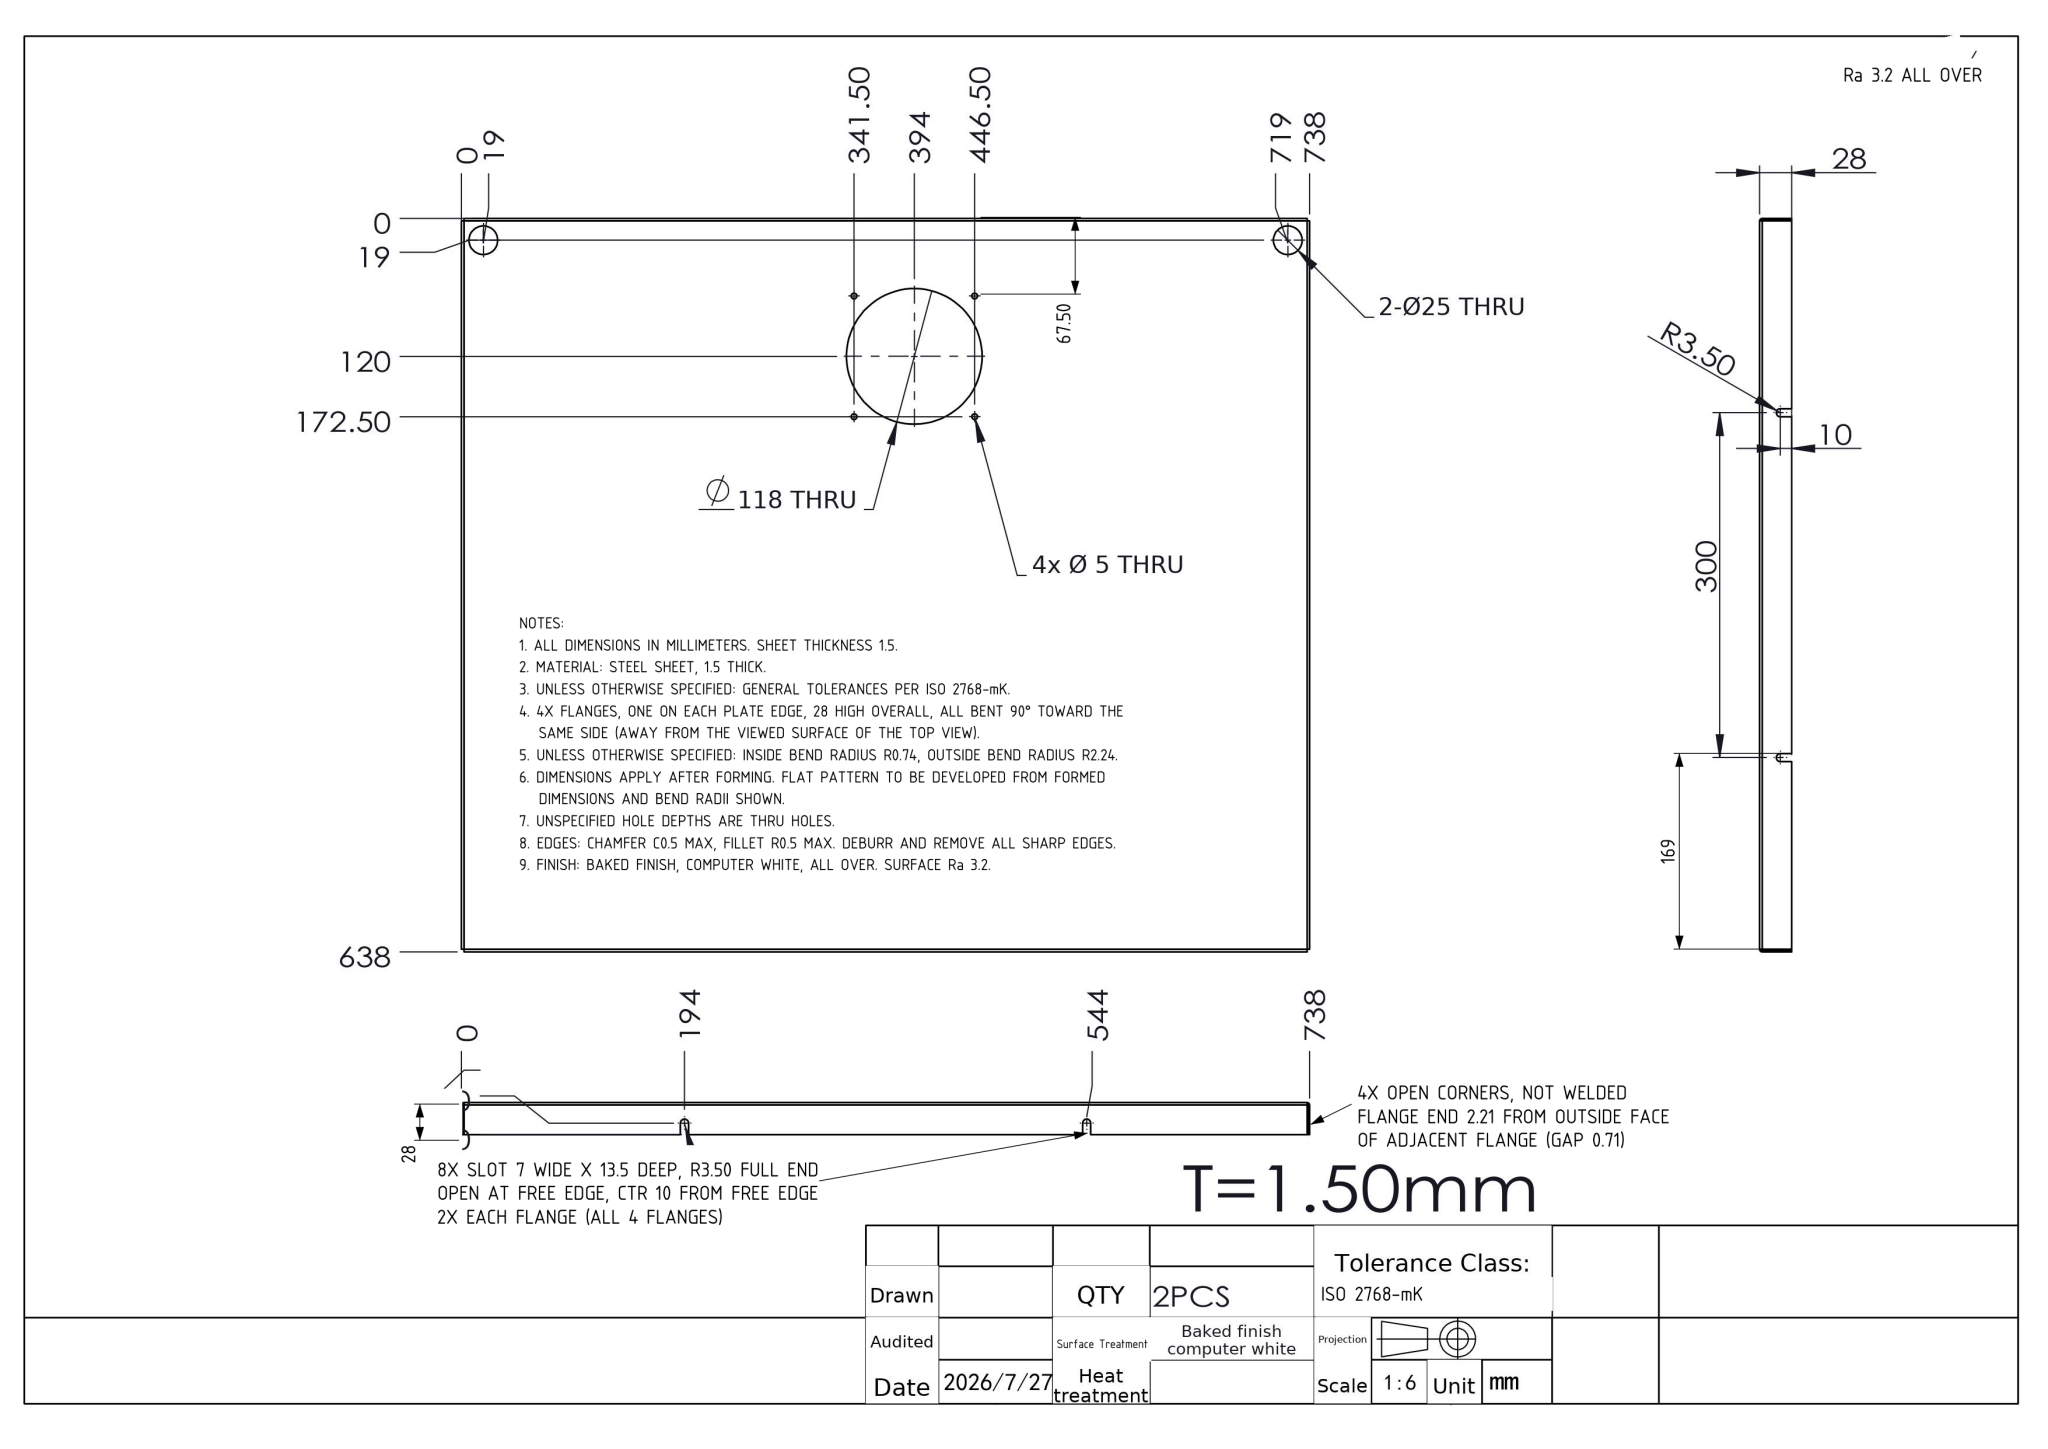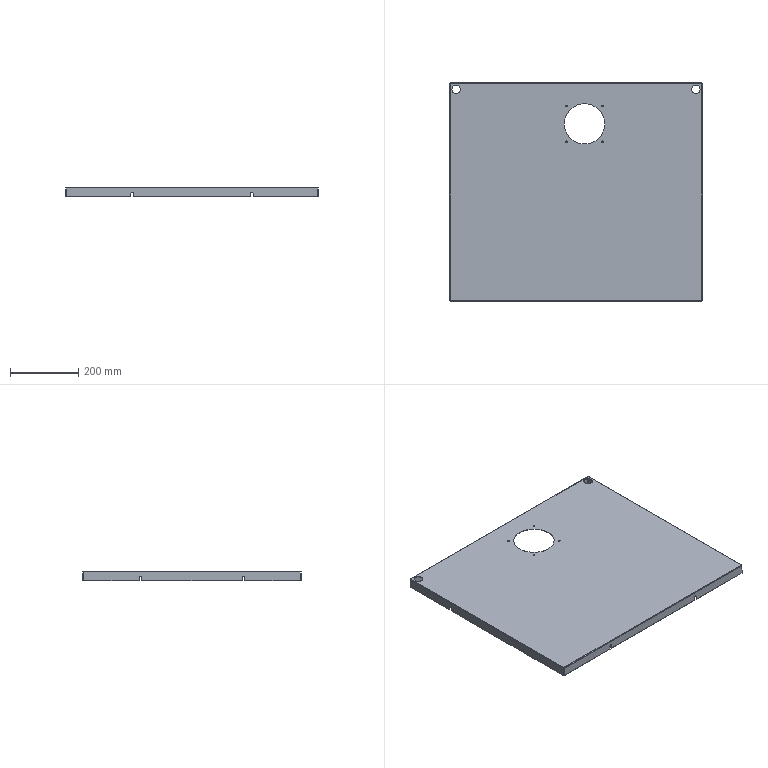Part | NX | mm | 1 solid | 84 faces | box 738 x 638 x 28 mm | volume 793245 mm3 | plane 46 | cylinder 30 | spline 8 | commonest cylinder face diameters 5 x8 7 x8 25 x4 4.473 x4 1.473 x4 118 x2